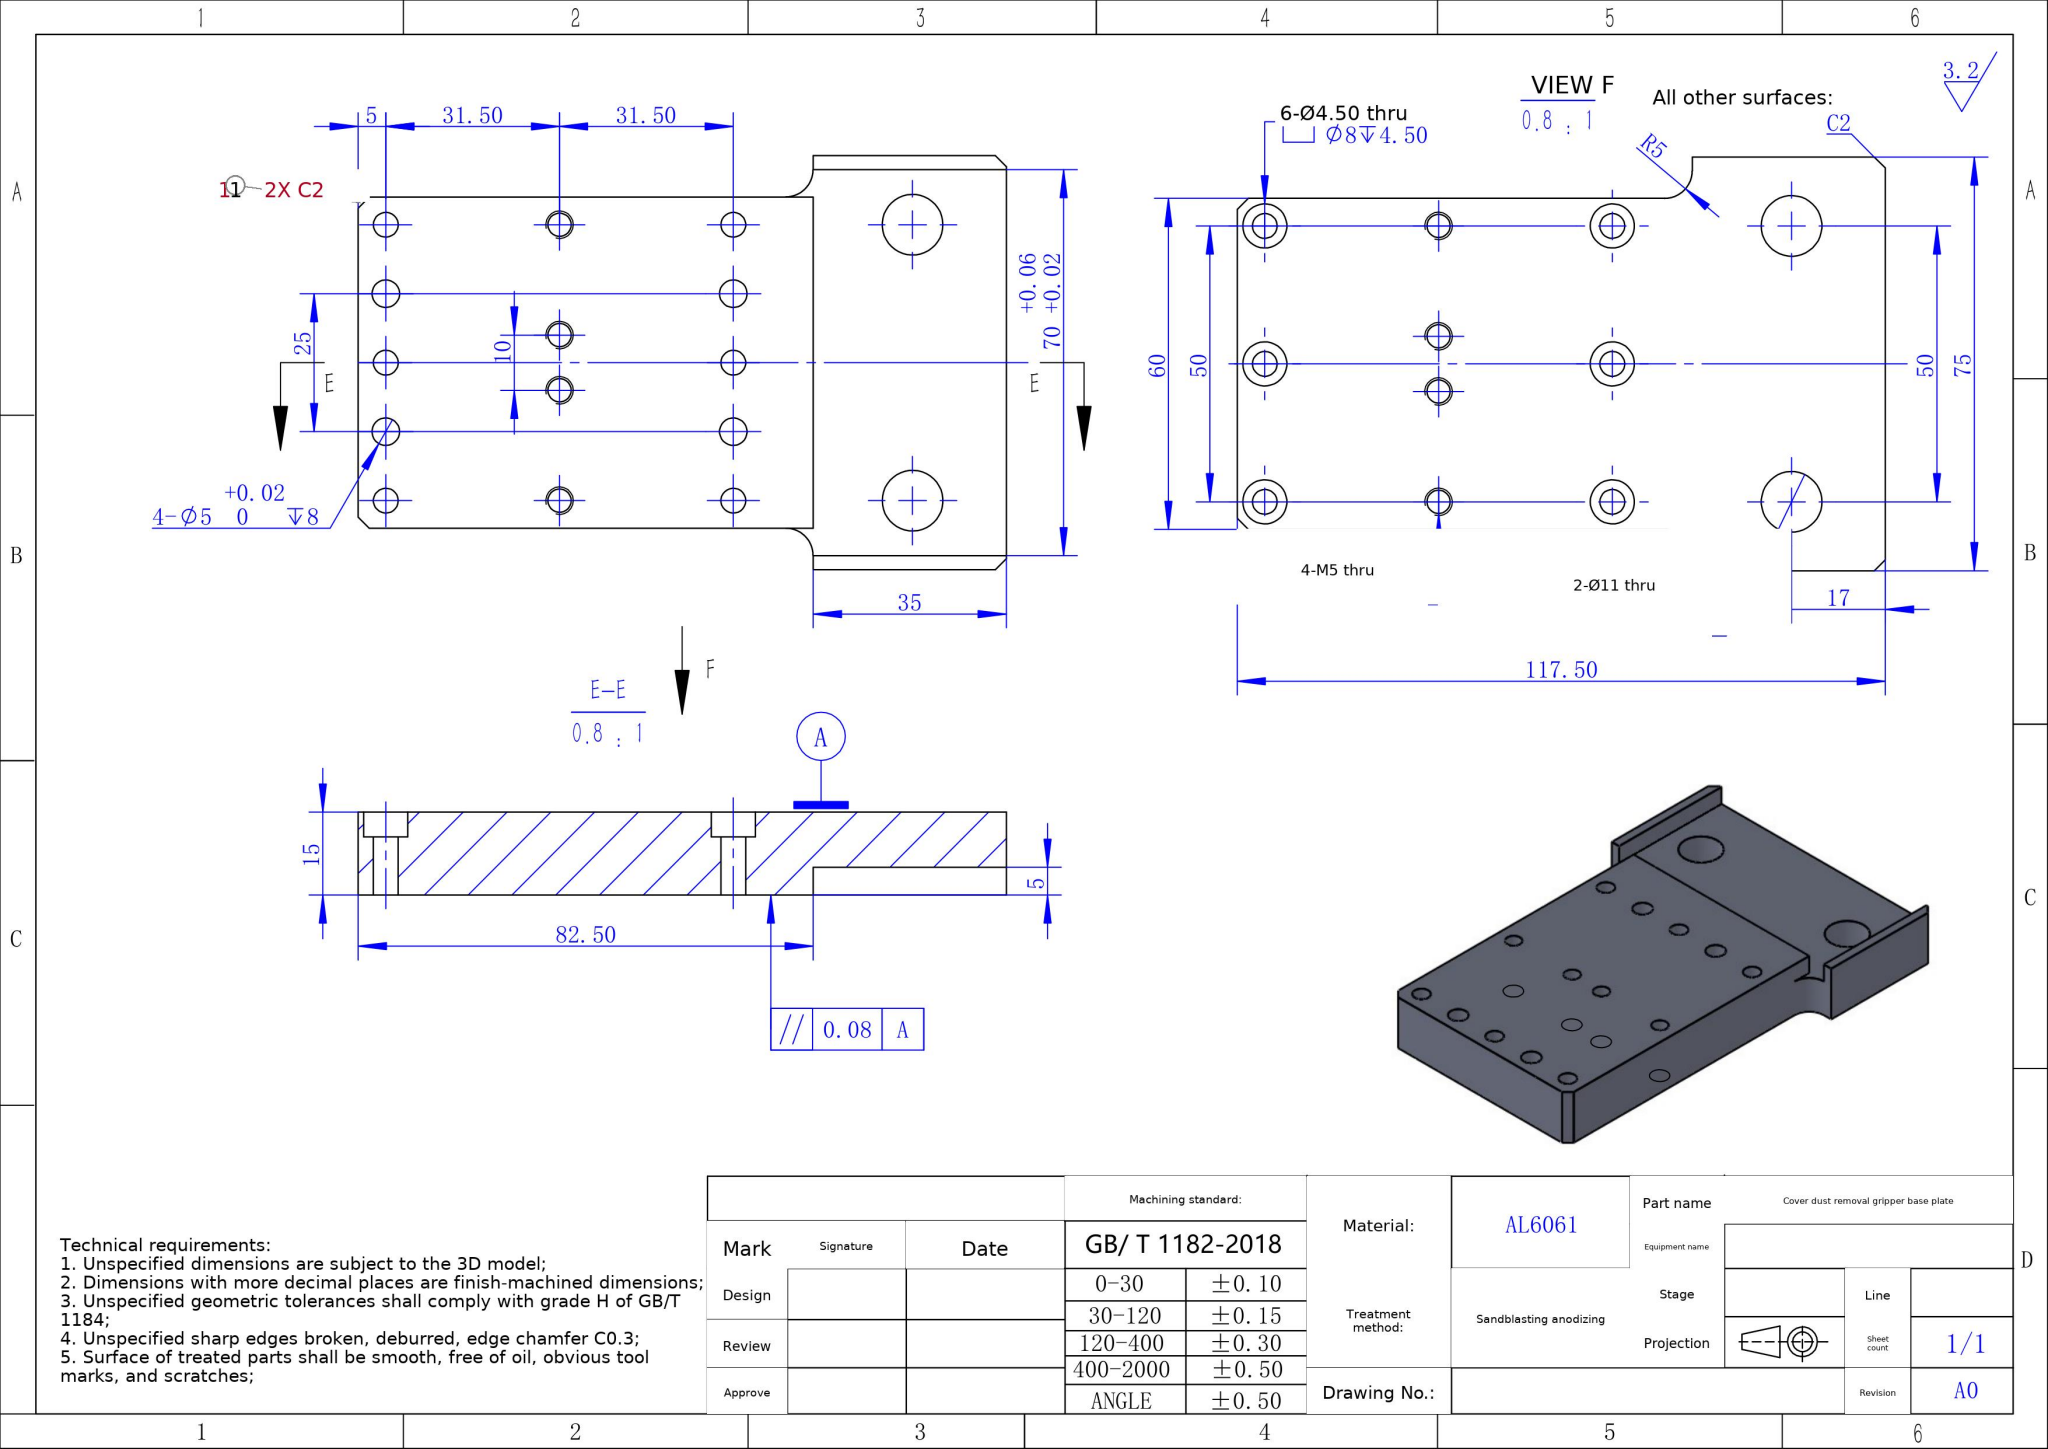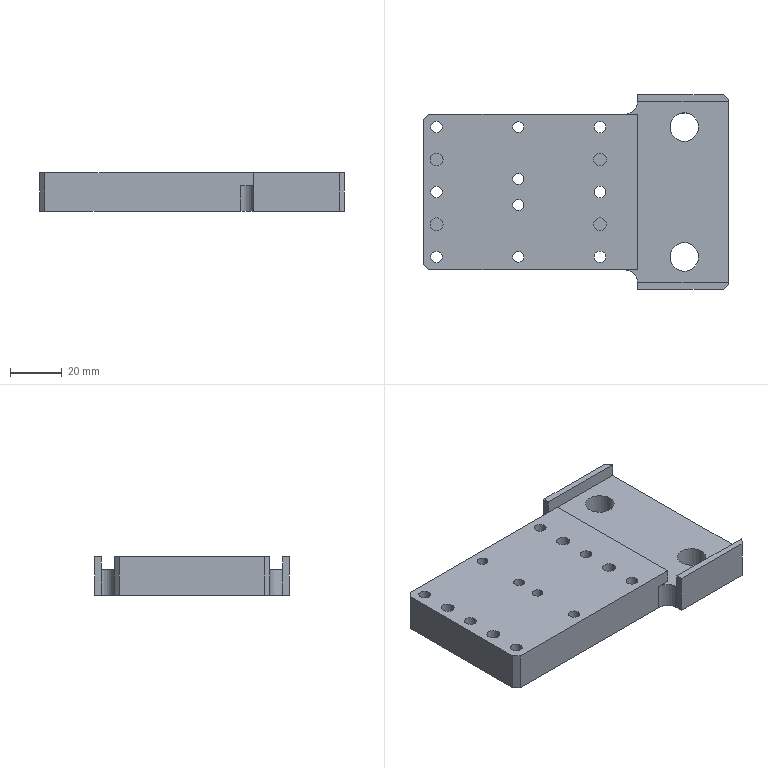Part | SolidWorks | mm | material AL6061 | 1 solid | 76 faces | box 117.5 x 75 x 15 mm | volume 95643 mm3 | cylinder 46 | plane 30 | commonest cylinder face diameters 8 x12 4.5 x12 4.2 x8 5 x8 11 x4 10 x2